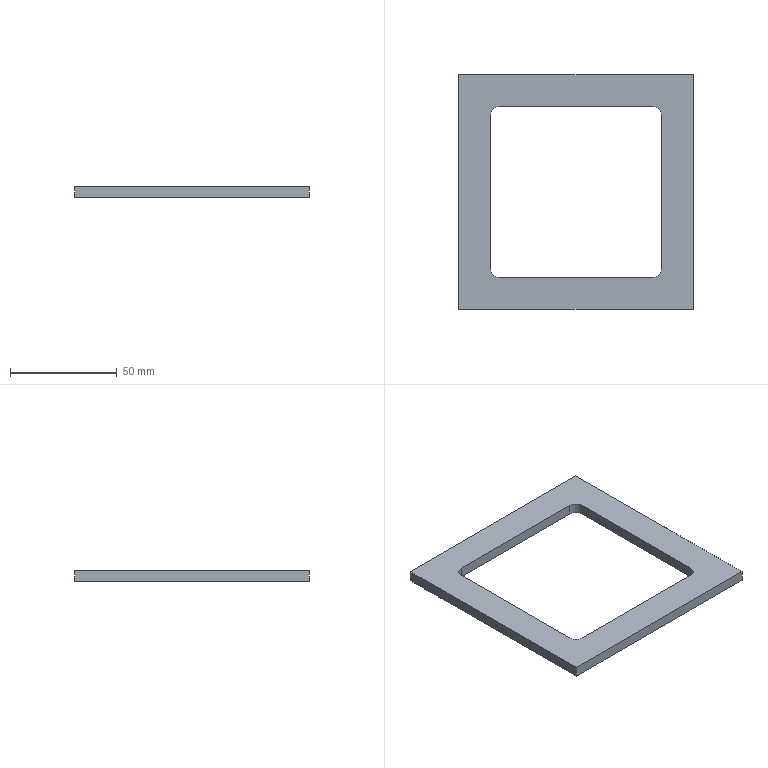Component | SolidWorks | YC1-250HangingBoxOverall-1_YC1-250SupportBracketT()-1_YC1-160BoxBaffleT-1 | 1 solid | 14 faces | box 110 x 110 x 5 mm | volume 28569 mm3 | plane 10 | cylinder 4 | commonest cylinder face diameters 8 x4 | material Plain Carbon Steel
STEP:
#1=COLOUR_RGB('',0.7922,0.8196,0.9333);
#2=FILL_AREA_STYLE_COLOUR('',#1);
#3=FILL_AREA_STYLE('',(#2));
#4=SURFACE_STYLE_FILL_AREA(#3);
#5=SURFACE_SIDE_STYLE('',(#4));
#6=SURFACE_STYLE_USAGE(.BOTH.,#5);
#7=PRESENTATION_STYLE_ASSIGNMENT((#6));
#8=CARTESIAN_POINT('',(33.268,60.906,-46.063));
#9=VERTEX_POINT('',#8);
#10=CARTESIAN_POINT('',(33.268,63.74,-46.063));
#11=VERTEX_POINT('',#10);
#12=CARTESIAN_POINT('',(33.268,64.488,-46.063));
#13=DIRECTION('',(0.,1.,0.));
#14=VECTOR('',#13,39.37);
#15=LINE('',#12,#14);
#16=EDGE_CURVE('',#9,#11,#15,.T.);
#17=ORIENTED_EDGE('',*,*,#16,.T.);
#18=CARTESIAN_POINT('',(33.11,63.898,-46.063));
#19=VERTEX_POINT('',#18);
#20=CARTESIAN_POINT('',(33.11,63.74,-46.063));
#21=DIRECTION('',(0.,0.,1.));
#22=DIRECTION('',(-1.,0.,0.));
#23=AXIS2_PLACEMENT_3D('',#20,#21,#22);
#24=CIRCLE('',#23,0.1575);
#25=EDGE_CURVE('',#11,#19,#24,.T.);
#26=ORIENTED_EDGE('',*,*,#25,.T.);
#27=CARTESIAN_POINT('',(30.276,63.898,-46.063));
#28=VERTEX_POINT('',#27);
#29=CARTESIAN_POINT('',(29.528,63.898,-46.063));
#30=DIRECTION('',(-1.,0.,0.));
#31=VECTOR('',#30,39.37);
#32=LINE('',#29,#31);
#33=EDGE_CURVE('',#19,#28,#32,.T.);
#34=ORIENTED_EDGE('',*,*,#33,.T.);
#35=CARTESIAN_POINT('',(30.118,63.74,-46.063));
#36=VERTEX_POINT('',#35);
#37=CARTESIAN_POINT('',(30.276,63.74,-46.063));
#38=DIRECTION('',(0.,0.,1.));
#39=DIRECTION('',(-1.,0.,0.));
#40=AXIS2_PLACEMENT_3D('',#37,#38,#39);
#41=CIRCLE('',#40,0.1575);
#42=EDGE_CURVE('',#28,#36,#41,.T.);
#43=ORIENTED_EDGE('',*,*,#42,.T.);
#44=CARTESIAN_POINT('',(30.118,60.906,-46.063));
#45=VERTEX_POINT('',#44);
#46=CARTESIAN_POINT('',(30.118,64.488,-46.063));
#47=DIRECTION('',(0.,-1.,0.));
#48=VECTOR('',#47,39.37);
#49=LINE('',#46,#48);
#50=EDGE_CURVE('',#36,#45,#49,.T.);
#51=ORIENTED_EDGE('',*,*,#50,.T.);
#52=CARTESIAN_POINT('',(30.276,60.748,-46.063));
#53=VERTEX_POINT('',#52);
#54=CARTESIAN_POINT('',(30.276,60.906,-46.063));
#55=DIRECTION('',(0.,0.,1.));
#56=DIRECTION('',(-1.,0.,0.));
#57=AXIS2_PLACEMENT_3D('',#54,#55,#56);
#58=CIRCLE('',#57,0.1575);
#59=EDGE_CURVE('',#45,#53,#58,.T.);
#60=ORIENTED_EDGE('',*,*,#59,.T.);
#61=CARTESIAN_POINT('',(33.11,60.748,-46.063));
#62=VERTEX_POINT('',#61);
#63=CARTESIAN_POINT('',(29.528,60.748,-46.063));
#64=DIRECTION('',(1.,0.,0.));
#65=VECTOR('',#64,39.37);
#66=LINE('',#63,#65);
#67=EDGE_CURVE('',#53,#62,#66,.T.);
#68=ORIENTED_EDGE('',*,*,#67,.T.);
#69=CARTESIAN_POINT('',(33.11,60.906,-46.063));
#70=DIRECTION('',(0.,0.,1.));
#71=DIRECTION('',(-1.,0.,0.));
#72=AXIS2_PLACEMENT_3D('',#69,#70,#71);
#73=CIRCLE('',#72,0.1575);
#74=EDGE_CURVE('',#62,#9,#73,.T.);
#75=ORIENTED_EDGE('',*,*,#74,.T.);
#76=EDGE_LOOP('',(#17,#26,#34,#43,#51,#60,#68,#75));
#77=FACE_BOUND('',#76,.T.);
#78=CARTESIAN_POINT('',(33.858,64.488,-46.063));
#79=VERTEX_POINT('',#78);
#80=CARTESIAN_POINT('',(33.858,60.157,-46.063));
#81=VERTEX_POINT('',#80);
#82=CARTESIAN_POINT('',(33.858,64.488,-46.063));
#83=DIRECTION('',(0.,-1.,0.));
#84=VECTOR('',#83,39.37);
#85=LINE('',#82,#84);
#86=EDGE_CURVE('',#79,#81,#85,.T.);
#87=ORIENTED_EDGE('',*,*,#86,.T.);
#88=CARTESIAN_POINT('',(29.528,60.157,-46.063));
#89=VERTEX_POINT('',#88);
#90=CARTESIAN_POINT('',(29.528,60.157,-46.063));
#91=DIRECTION('',(-1.,0.,0.));
#92=VECTOR('',#91,39.37);
#93=LINE('',#90,#92);
#94=EDGE_CURVE('',#81,#89,#93,.T.);
#95=ORIENTED_EDGE('',*,*,#94,.T.);
#96=CARTESIAN_POINT('',(29.528,64.488,-46.063));
#97=VERTEX_POINT('',#96);
#98=CARTESIAN_POINT('',(29.528,64.488,-46.063));
#99=DIRECTION('',(0.,1.,0.));
#100=VECTOR('',#99,39.37);
#101=LINE('',#98,#100);
#102=EDGE_CURVE('',#89,#97,#101,.T.);
#103=ORIENTED_EDGE('',*,*,#102,.T.);
#104=CARTESIAN_POINT('',(29.528,64.488,-46.063));
#105=DIRECTION('',(1.,0.,0.));
#106=VECTOR('',#105,39.37);
#107=LINE('',#104,#106);
#108=EDGE_CURVE('',#97,#79,#107,.T.);
#109=ORIENTED_EDGE('',*,*,#108,.T.);
#110=EDGE_LOOP('',(#87,#95,#103,#109));
#111=FACE_OUTER_BOUND('',#110,.T.);
#112=CARTESIAN_POINT('',(29.528,64.488,-46.063));
#113=DIRECTION('',(0.,0.,-1.));
#114=DIRECTION('',(-1.,0.,0.));
#115=AXIS2_PLACEMENT_3D('',#112,#113,#114);
#116=PLANE('',#115);
#117=ADVANCED_FACE('',(#77,#111),#116,.T.);
#118=CARTESIAN_POINT('',(33.268,63.74,-45.866));
#119=VERTEX_POINT('',#118);
#120=CARTESIAN_POINT('',(33.268,63.74,-45.866));
#121=DIRECTION('',(0.,0.,-1.));
#122=VECTOR('',#121,39.37);
#123=LINE('',#120,#122);
#124=EDGE_CURVE('',#119,#11,#123,.T.);
#125=ORIENTED_EDGE('',*,*,#124,.F.);
#126=CARTESIAN_POINT('',(33.11,63.898,-45.866));
#127=VERTEX_POINT('',#126);
#128=CARTESIAN_POINT('',(33.11,63.74,-45.866));
#129=DIRECTION('',(0.,0.,-1.));
#130=DIRECTION('',(-1.,0.,0.));
#131=AXIS2_PLACEMENT_3D('',#128,#129,#130);
#132=CIRCLE('',#131,0.1575);
#133=EDGE_CURVE('',#127,#119,#132,.T.);
#134=ORIENTED_EDGE('',*,*,#133,.F.);
#135=CARTESIAN_POINT('',(33.11,63.898,-45.866));
#136=DIRECTION('',(0.,0.,1.));
#137=VECTOR('',#136,39.37);
#138=LINE('',#135,#137);
#139=EDGE_CURVE('',#19,#127,#138,.T.);
#140=ORIENTED_EDGE('',*,*,#139,.F.);
#141=ORIENTED_EDGE('',*,*,#25,.F.);
#142=EDGE_LOOP('',(#125,#134,#140,#141));
#143=FACE_OUTER_BOUND('',#142,.T.);
#144=CARTESIAN_POINT('',(33.11,63.74,-45.866));
#145=DIRECTION('',(0.,0.,-1.));
#146=DIRECTION('',(-1.,0.,0.));
#147=AXIS2_PLACEMENT_3D('',#144,#145,#146);
#148=CYLINDRICAL_SURFACE('',#147,0.1575);
#149=ADVANCED_FACE('',(#143),#148,.F.);
#150=CARTESIAN_POINT('',(33.268,60.906,-45.866));
#151=VERTEX_POINT('',#150);
#152=CARTESIAN_POINT('',(33.268,60.906,-45.866));
#153=DIRECTION('',(0.,1.,0.));
#154=VECTOR('',#153,39.37);
#155=LINE('',#152,#154);
#156=EDGE_CURVE('',#151,#119,#155,.T.);
#157=ORIENTED_EDGE('',*,*,#156,.T.);
#158=ORIENTED_EDGE('',*,*,#124,.T.);
#159=ORIENTED_EDGE('',*,*,#16,.F.);
#160=CARTESIAN_POINT('',(33.268,60.906,-45.866));
#161=DIRECTION('',(0.,0.,1.));
#162=VECTOR('',#161,39.37);
#163=LINE('',#160,#162);
#164=EDGE_CURVE('',#9,#151,#163,.T.);
#165=ORIENTED_EDGE('',*,*,#164,.T.);
#166=EDGE_LOOP('',(#157,#158,#159,#165));
#167=FACE_OUTER_BOUND('',#166,.T.);
#168=CARTESIAN_POINT('',(33.268,60.906,-45.866));
#169=DIRECTION('',(-1.,0.,0.));
#170=DIRECTION('',(0.,0.,1.));
#171=AXIS2_PLACEMENT_3D('',#168,#169,#170);
#172=PLANE('',#171);
#173=ADVANCED_FACE('',(#167),#172,.T.);
#174=CARTESIAN_POINT('',(33.11,60.748,-45.866));
#175=VERTEX_POINT('',#174);
#176=CARTESIAN_POINT('',(33.11,60.748,-45.866));
#177=DIRECTION('',(0.,0.,-1.));
#178=VECTOR('',#177,39.37);
#179=LINE('',#176,#178);
#180=EDGE_CURVE('',#175,#62,#179,.T.);
#181=ORIENTED_EDGE('',*,*,#180,.F.);
#182=CARTESIAN_POINT('',(33.11,60.906,-45.866));
#183=DIRECTION('',(0.,0.,-1.));
#184=DIRECTION('',(-1.,0.,0.));
#185=AXIS2_PLACEMENT_3D('',#182,#183,#184);
#186=CIRCLE('',#185,0.1575);
#187=EDGE_CURVE('',#151,#175,#186,.T.);
#188=ORIENTED_EDGE('',*,*,#187,.F.);
#189=ORIENTED_EDGE('',*,*,#164,.F.);
#190=ORIENTED_EDGE('',*,*,#74,.F.);
#191=EDGE_LOOP('',(#181,#188,#189,#190));
#192=FACE_OUTER_BOUND('',#191,.T.);
#193=CARTESIAN_POINT('',(33.11,60.906,-45.866));
#194=DIRECTION('',(0.,0.,-1.));
#195=DIRECTION('',(-1.,0.,0.));
#196=AXIS2_PLACEMENT_3D('',#193,#194,#195);
#197=CYLINDRICAL_SURFACE('',#196,0.1575);
#198=ADVANCED_FACE('',(#192),#197,.F.);
#199=CARTESIAN_POINT('',(30.276,60.748,-45.866));
#200=VERTEX_POINT('',#199);
#201=CARTESIAN_POINT('',(30.276,60.748,-45.866));
#202=DIRECTION('',(1.,0.,0.));
#203=VECTOR('',#202,39.37);
#204=LINE('',#201,#203);
#205=EDGE_CURVE('',#200,#175,#204,.T.);
#206=ORIENTED_EDGE('',*,*,#205,.T.);
#207=ORIENTED_EDGE('',*,*,#180,.T.);
#208=ORIENTED_EDGE('',*,*,#67,.F.);
#209=CARTESIAN_POINT('',(30.276,60.748,-45.866));
#210=DIRECTION('',(0.,0.,1.));
#211=VECTOR('',#210,39.37);
#212=LINE('',#209,#211);
#213=EDGE_CURVE('',#53,#200,#212,.T.);
#214=ORIENTED_EDGE('',*,*,#213,.T.);
#215=EDGE_LOOP('',(#206,#207,#208,#214));
#216=FACE_OUTER_BOUND('',#215,.T.);
#217=CARTESIAN_POINT('',(30.276,60.748,-45.866));
#218=DIRECTION('',(0.,1.,0.));
#219=DIRECTION('',(0.,0.,1.));
#220=AXIS2_PLACEMENT_3D('',#217,#218,#219);
#221=PLANE('',#220);
#222=ADVANCED_FACE('',(#216),#221,.T.);
#223=CARTESIAN_POINT('',(30.118,60.906,-45.866));
#224=VERTEX_POINT('',#223);
#225=CARTESIAN_POINT('',(30.118,60.906,-45.866));
#226=DIRECTION('',(0.,0.,-1.));
#227=VECTOR('',#226,39.37);
#228=LINE('',#225,#227);
#229=EDGE_CURVE('',#224,#45,#228,.T.);
#230=ORIENTED_EDGE('',*,*,#229,.F.);
#231=CARTESIAN_POINT('',(30.276,60.906,-45.866));
#232=DIRECTION('',(0.,0.,-1.));
#233=DIRECTION('',(-1.,0.,0.));
#234=AXIS2_PLACEMENT_3D('',#231,#232,#233);
#235=CIRCLE('',#234,0.1575);
#236=EDGE_CURVE('',#200,#224,#235,.T.);
#237=ORIENTED_EDGE('',*,*,#236,.F.);
#238=ORIENTED_EDGE('',*,*,#213,.F.);
#239=ORIENTED_EDGE('',*,*,#59,.F.);
#240=EDGE_LOOP('',(#230,#237,#238,#239));
#241=FACE_OUTER_BOUND('',#240,.T.);
#242=CARTESIAN_POINT('',(30.276,60.906,-45.866));
#243=DIRECTION('',(0.,0.,-1.));
#244=DIRECTION('',(-1.,0.,0.));
#245=AXIS2_PLACEMENT_3D('',#242,#243,#244);
#246=CYLINDRICAL_SURFACE('',#245,0.1575);
#247=ADVANCED_FACE('',(#241),#246,.F.);
#248=CARTESIAN_POINT('',(30.118,63.74,-45.866));
#249=VERTEX_POINT('',#248);
#250=CARTESIAN_POINT('',(30.118,60.906,-45.866));
#251=DIRECTION('',(0.,-1.,0.));
#252=VECTOR('',#251,39.37);
#253=LINE('',#250,#252);
#254=EDGE_CURVE('',#249,#224,#253,.T.);
#255=ORIENTED_EDGE('',*,*,#254,.T.);
#256=ORIENTED_EDGE('',*,*,#229,.T.);
#257=ORIENTED_EDGE('',*,*,#50,.F.);
#258=CARTESIAN_POINT('',(30.118,63.74,-45.866));
#259=DIRECTION('',(0.,0.,1.));
#260=VECTOR('',#259,39.37);
#261=LINE('',#258,#260);
#262=EDGE_CURVE('',#36,#249,#261,.T.);
#263=ORIENTED_EDGE('',*,*,#262,.T.);
#264=EDGE_LOOP('',(#255,#256,#257,#263));
#265=FACE_OUTER_BOUND('',#264,.T.);
#266=CARTESIAN_POINT('',(30.118,60.906,-45.866));
#267=DIRECTION('',(1.,0.,0.));
#268=DIRECTION('',(0.,0.,-1.));
#269=AXIS2_PLACEMENT_3D('',#266,#267,#268);
#270=PLANE('',#269);
#271=ADVANCED_FACE('',(#265),#270,.T.);
#272=CARTESIAN_POINT('',(30.276,63.898,-45.866));
#273=VERTEX_POINT('',#272);
#274=CARTESIAN_POINT('',(30.276,63.898,-45.866));
#275=DIRECTION('',(0.,0.,-1.));
#276=VECTOR('',#275,39.37);
#277=LINE('',#274,#276);
#278=EDGE_CURVE('',#273,#28,#277,.T.);
#279=ORIENTED_EDGE('',*,*,#278,.F.);
#280=CARTESIAN_POINT('',(30.276,63.74,-45.866));
#281=DIRECTION('',(0.,0.,-1.));
#282=DIRECTION('',(-1.,0.,0.));
#283=AXIS2_PLACEMENT_3D('',#280,#281,#282);
#284=CIRCLE('',#283,0.1575);
#285=EDGE_CURVE('',#249,#273,#284,.T.);
#286=ORIENTED_EDGE('',*,*,#285,.F.);
#287=ORIENTED_EDGE('',*,*,#262,.F.);
#288=ORIENTED_EDGE('',*,*,#42,.F.);
#289=EDGE_LOOP('',(#279,#286,#287,#288));
#290=FACE_OUTER_BOUND('',#289,.T.);
#291=CARTESIAN_POINT('',(30.276,63.74,-45.866));
#292=DIRECTION('',(0.,0.,-1.));
#293=DIRECTION('',(-1.,0.,0.));
#294=AXIS2_PLACEMENT_3D('',#291,#292,#293);
#295=CYLINDRICAL_SURFACE('',#294,0.1575);
#296=ADVANCED_FACE('',(#290),#295,.F.);
#297=CARTESIAN_POINT('',(30.276,63.898,-45.866));
#298=DIRECTION('',(-1.,0.,0.));
#299=VECTOR('',#298,39.37);
#300=LINE('',#297,#299);
#301=EDGE_CURVE('',#127,#273,#300,.T.);
#302=ORIENTED_EDGE('',*,*,#301,.T.);
#303=ORIENTED_EDGE('',*,*,#278,.T.);
#304=ORIENTED_EDGE('',*,*,#33,.F.);
#305=ORIENTED_EDGE('',*,*,#139,.T.);
#306=EDGE_LOOP('',(#302,#303,#304,#305));
#307=FACE_OUTER_BOUND('',#306,.T.);
#308=CARTESIAN_POINT('',(30.276,63.898,-45.866));
#309=DIRECTION('',(0.,-1.,0.));
#310=DIRECTION('',(0.,0.,-1.));
#311=AXIS2_PLACEMENT_3D('',#308,#309,#310);
#312=PLANE('',#311);
#313=ADVANCED_FACE('',(#307),#312,.T.);
#314=CARTESIAN_POINT('',(33.858,60.157,-45.866));
#315=VERTEX_POINT('',#314);
#316=CARTESIAN_POINT('',(33.858,60.157,-45.866));
#317=DIRECTION('',(0.,0.,-1.));
#318=VECTOR('',#317,39.37);
#319=LINE('',#316,#318);
#320=EDGE_CURVE('',#315,#81,#319,.T.);
#321=ORIENTED_EDGE('',*,*,#320,.F.);
#322=CARTESIAN_POINT('',(29.528,60.157,-45.866));
#323=VERTEX_POINT('',#322);
#324=CARTESIAN_POINT('',(29.528,60.157,-45.866));
#325=DIRECTION('',(1.,0.,0.));
#326=VECTOR('',#325,39.37);
#327=LINE('',#324,#326);
#328=EDGE_CURVE('',#323,#315,#327,.T.);
#329=ORIENTED_EDGE('',*,*,#328,.F.);
#330=CARTESIAN_POINT('',(29.528,60.157,-45.866));
#331=DIRECTION('',(0.,0.,1.));
#332=VECTOR('',#331,39.37);
#333=LINE('',#330,#332);
#334=EDGE_CURVE('',#89,#323,#333,.T.);
#335=ORIENTED_EDGE('',*,*,#334,.F.);
#336=ORIENTED_EDGE('',*,*,#94,.F.);
#337=EDGE_LOOP('',(#321,#329,#335,#336));
#338=FACE_OUTER_BOUND('',#337,.T.);
#339=CARTESIAN_POINT('',(29.528,60.157,-45.866));
#340=DIRECTION('',(0.,1.,0.));
#341=DIRECTION('',(0.,0.,1.));
#342=AXIS2_PLACEMENT_3D('',#339,#340,#341);
#343=PLANE('',#342);
#344=ADVANCED_FACE('',(#338),#343,.F.);
#345=CARTESIAN_POINT('',(33.858,64.488,-45.866));
#346=VERTEX_POINT('',#345);
#347=CARTESIAN_POINT('',(33.858,64.488,-45.866));
#348=DIRECTION('',(0.,0.,-1.));
#349=VECTOR('',#348,39.37);
#350=LINE('',#347,#349);
#351=EDGE_CURVE('',#346,#79,#350,.T.);
#352=ORIENTED_EDGE('',*,*,#351,.F.);
#353=CARTESIAN_POINT('',(33.858,60.157,-45.866));
#354=DIRECTION('',(0.,1.,0.));
#355=VECTOR('',#354,39.37);
#356=LINE('',#353,#355);
#357=EDGE_CURVE('',#315,#346,#356,.T.);
#358=ORIENTED_EDGE('',*,*,#357,.F.);
#359=ORIENTED_EDGE('',*,*,#320,.T.);
#360=ORIENTED_EDGE('',*,*,#86,.F.);
#361=EDGE_LOOP('',(#352,#358,#359,#360));
#362=FACE_OUTER_BOUND('',#361,.T.);
#363=CARTESIAN_POINT('',(33.858,60.157,-45.866));
#364=DIRECTION('',(-1.,0.,0.));
#365=DIRECTION('',(0.,0.,1.));
#366=AXIS2_PLACEMENT_3D('',#363,#364,#365);
#367=PLANE('',#366);
#368=ADVANCED_FACE('',(#362),#367,.F.);
#369=CARTESIAN_POINT('',(29.528,64.488,-45.866));
#370=VERTEX_POINT('',#369);
#371=CARTESIAN_POINT('',(29.528,64.488,-45.866));
#372=DIRECTION('',(0.,0.,-1.));
#373=VECTOR('',#372,39.37);
#374=LINE('',#371,#373);
#375=EDGE_CURVE('',#370,#97,#374,.T.);
#376=ORIENTED_EDGE('',*,*,#375,.F.);
#377=CARTESIAN_POINT('',(29.528,64.488,-45.866));
#378=DIRECTION('',(-1.,0.,0.));
#379=VECTOR('',#378,39.37);
#380=LINE('',#377,#379);
#381=EDGE_CURVE('',#346,#370,#380,.T.);
#382=ORIENTED_EDGE('',*,*,#381,.F.);
#383=ORIENTED_EDGE('',*,*,#351,.T.);
#384=ORIENTED_EDGE('',*,*,#108,.F.);
#385=EDGE_LOOP('',(#376,#382,#383,#384));
#386=FACE_OUTER_BOUND('',#385,.T.);
#387=CARTESIAN_POINT('',(29.528,64.488,-45.866));
#388=DIRECTION('',(0.,-1.,0.));
#389=DIRECTION('',(0.,0.,-1.));
#390=AXIS2_PLACEMENT_3D('',#387,#388,#389);
#391=PLANE('',#390);
#392=ADVANCED_FACE('',(#386),#391,.F.);
#393=ORIENTED_EDGE('',*,*,#334,.T.);
#394=CARTESIAN_POINT('',(29.528,60.157,-45.866));
#395=DIRECTION('',(0.,-1.,0.));
#396=VECTOR('',#395,39.37);
#397=LINE('',#394,#396);
#398=EDGE_CURVE('',#370,#323,#397,.T.);
#399=ORIENTED_EDGE('',*,*,#398,.F.);
#400=ORIENTED_EDGE('',*,*,#375,.T.);
#401=ORIENTED_EDGE('',*,*,#102,.F.);
#402=EDGE_LOOP('',(#393,#399,#400,#401));
#403=FACE_OUTER_BOUND('',#402,.T.);
#404=CARTESIAN_POINT('',(29.528,60.157,-45.866));
#405=DIRECTION('',(1.,0.,0.));
#406=DIRECTION('',(0.,0.,-1.));
#407=AXIS2_PLACEMENT_3D('',#404,#405,#406);
#408=PLANE('',#407);
#409=ADVANCED_FACE('',(#403),#408,.F.);
#410=ORIENTED_EDGE('',*,*,#301,.F.);
#411=ORIENTED_EDGE('',*,*,#133,.T.);
#412=ORIENTED_EDGE('',*,*,#156,.F.);
#413=ORIENTED_EDGE('',*,*,#187,.T.);
#414=ORIENTED_EDGE('',*,*,#205,.F.);
#415=ORIENTED_EDGE('',*,*,#236,.T.);
#416=ORIENTED_EDGE('',*,*,#254,.F.);
#417=ORIENTED_EDGE('',*,*,#285,.T.);
#418=EDGE_LOOP('',(#410,#411,#412,#413,#414,#415,#416,#417));
#419=FACE_BOUND('',#418,.T.);
#420=ORIENTED_EDGE('',*,*,#328,.T.);
#421=ORIENTED_EDGE('',*,*,#357,.T.);
#422=ORIENTED_EDGE('',*,*,#381,.T.);
#423=ORIENTED_EDGE('',*,*,#398,.T.);
#424=EDGE_LOOP('',(#420,#421,#422,#423));
#425=FACE_OUTER_BOUND('',#424,.T.);
#426=CARTESIAN_POINT('',(29.528,64.488,-45.866));
#427=DIRECTION('',(0.,0.,-1.));
#428=DIRECTION('',(-1.,0.,0.));
#429=AXIS2_PLACEMENT_3D('',#426,#427,#428);
#430=PLANE('',#429);
#431=ADVANCED_FACE('',(#419,#425),#430,.F.);
#432=CLOSED_SHELL('',(#117,#149,#173,#198,#222,#247,#271,#296,#313,#344,#368,#392,#409,#431));
#433=MANIFOLD_SOLID_BREP('',#432);
#434=STYLED_ITEM('',(#7),#433);
#435=(LENGTH_UNIT()NAMED_UNIT(*)SI_UNIT($,.METRE.));
#436=LENGTH_MEASURE_WITH_UNIT(LENGTH_MEASURE(0.0254),#435);
#437=DIMENSIONAL_EXPONENTS(1.,0.,0.,0.,0.,0.,0.);
#438=(CONVERSION_BASED_UNIT('',#436)LENGTH_UNIT()NAMED_UNIT(#437));
#439=UNCERTAINTY_MEASURE_WITH_UNIT(LENGTH_MEASURE(0.00001),#438,'','');
#440=(NAMED_UNIT(*)PLANE_ANGLE_UNIT()SI_UNIT($,.RADIAN.));
#441=(NAMED_UNIT(*)SI_UNIT($,.STERADIAN.)SOLID_ANGLE_UNIT());
#442=(GEOMETRIC_REPRESENTATION_CONTEXT(3)GLOBAL_UNCERTAINTY_ASSIGNED_CONTEXT((#439))GLOBAL_UNIT_ASSIGNED_CONTEXT((#438,#440,#441))REPRESENTATION_CONTEXT('',''));
#443=MECHANICAL_DESIGN_GEOMETRIC_PRESENTATION_REPRESENTATION('',(#434),#442);
#444=PRESENTATION_LAYER_ASSIGNMENT('','',(#434));
#445=CARTESIAN_POINT('',(0.,0.,0.));
#446=DIRECTION('',(0.,0.,1.));
#447=DIRECTION('',(1.,0.,0.));
#448=AXIS2_PLACEMENT_3D('',#445,#446,#447);
#449=(LENGTH_UNIT()NAMED_UNIT(*)SI_UNIT($,.METRE.));
#450=LENGTH_MEASURE_WITH_UNIT(LENGTH_MEASURE(0.0254),#449);
#451=DIMENSIONAL_EXPONENTS(1.,0.,0.,0.,0.,0.,0.);
#452=(CONVERSION_BASED_UNIT('',#450)LENGTH_UNIT()NAMED_UNIT(#451));
#453=UNCERTAINTY_MEASURE_WITH_UNIT(LENGTH_MEASURE(0.00001),#452,'','');
#454=(NAMED_UNIT(*)PLANE_ANGLE_UNIT()SI_UNIT($,.RADIAN.));
#455=(NAMED_UNIT(*)SI_UNIT($,.STERADIAN.)SOLID_ANGLE_UNIT());
#456=(GEOMETRIC_REPRESENTATION_CONTEXT(3)GLOBAL_UNCERTAINTY_ASSIGNED_CONTEXT((#453))GLOBAL_UNIT_ASSIGNED_CONTEXT((#452,#454,#455))REPRESENTATION_CONTEXT('',''));
#457=ADVANCED_BREP_SHAPE_REPRESENTATION('',(#433,#448),#456);